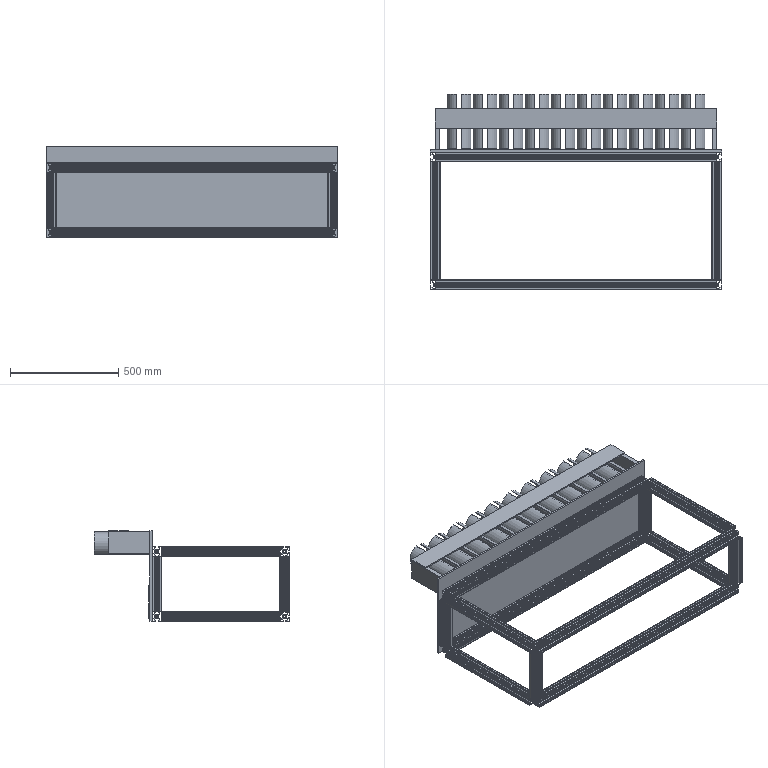Component | SolidWorks | FeedingMechanism-1 | 40 solids | 1788 faces | volume 16337143 mm3 | plane 1544 | cylinder 244 | commonest cylinder face diameters 10 x108 3 x48 5 x48 110 x20 100 x20